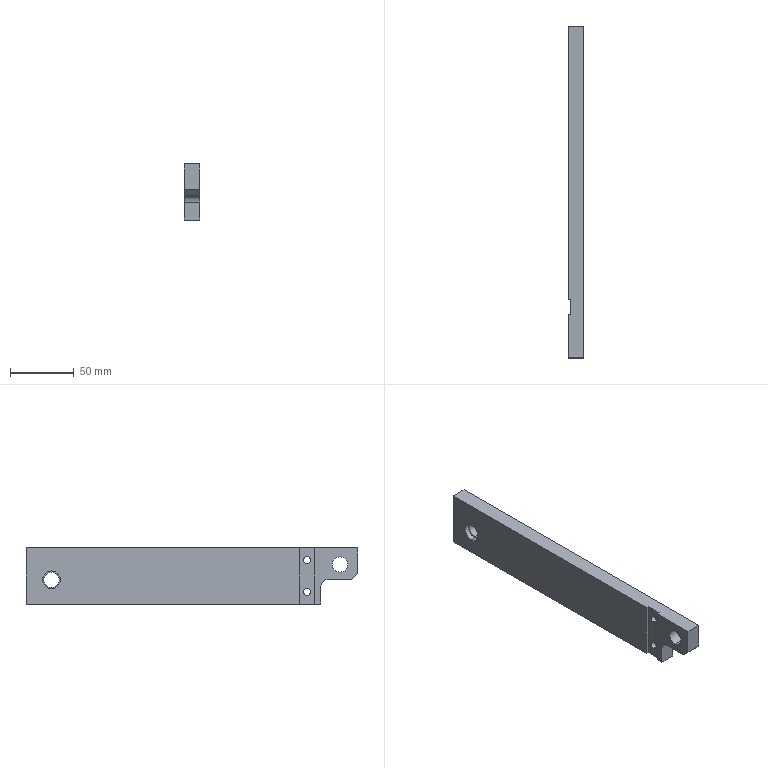Component | SolidWorks | STB-08-042JX-1 | 1 solid | 47 faces | volume 124834 mm3 | cylinder 23 | plane 16 | cone 8 | commonest cylinder face diameters 10 x5 12 x4 3.3 x4 5.5 x4 4.2 x4 14 x2 | material 6061 Alloy